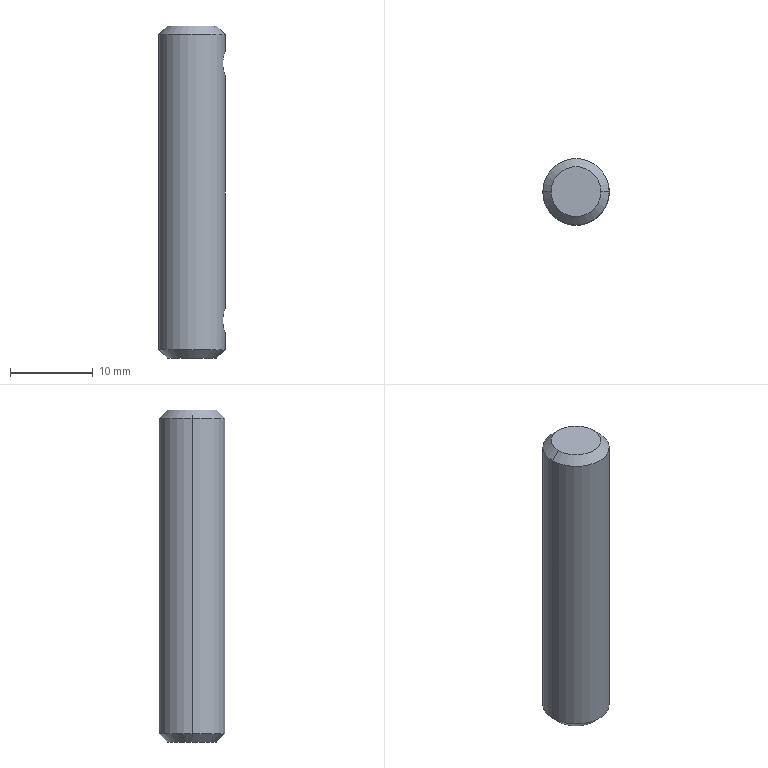Component | SolidWorks | ZTDJ-L-400-04-25-MaterialPortBagClamp-Axis6-1 | 1 solid | 16 faces | box 8 x 8 x 40 mm | volume 1928 mm3 | cone 8 | cylinder 6 | plane 2 | commonest cylinder face diameters 3 x4 8 x2 | material Alloy Steel
build123d program:
from build123d import *

# Parameters (mm, degrees)
SKETCH1_R                    = 4
BOSS_EXTRUDE1_DEPTH          = 20
F_3_0_3_DIAMETER_HOLE1_D     = 3
F_3_0_3_DIAMETER_HOLE1_DEPTH = 4
F_3_0_3_DIAMETER_HOLE1_TIP   = 0.9013
CHAMFER1_SIZE                = 1


with BuildPart() as part:
    # Sketch1 → Boss-Extrude1 (new, symmetric)
    with BuildSketch(Plane.XY):
        Circle(SKETCH1_R)
    extrude(amount=BOSS_EXTRUDE1_DEPTH, both=True)

    # 3.0 _3_ Diameter Hole1
    with Locations(Plane(origin=(4, 0, 0), x_dir=(0, 0, -1), z_dir=(1, 0, 0))):
        with Locations((-15.5, 0), (15.5, 0)):
            Hole(F_3_0_3_DIAMETER_HOLE1_D / 2, depth=F_3_0_3_DIAMETER_HOLE1_DEPTH)
            with Locations((0, 0, -(F_3_0_3_DIAMETER_HOLE1_DEPTH + F_3_0_3_DIAMETER_HOLE1_TIP / 2))):  # 118° drill point
                Cone(0, F_3_0_3_DIAMETER_HOLE1_D / 2, F_3_0_3_DIAMETER_HOLE1_TIP, mode=Mode.SUBTRACT)

    # Chamfer1
    chamfer1_edges = [part.edges().sort_by_distance(p)[0] for p in [
        (-4, 0, -20),
        (-4, 0, 20),
    ]]
    chamfer(chamfer1_edges, length=CHAMFER1_SIZE)


solid = part.part

# Placed as in the assembly
solid = solid.moved(Location((14.378, -64.673, 290), (0, 0, 0)))
STEP:
#1=COLOUR_RGB('',0.7922,0.8196,0.9333);
#2=FILL_AREA_STYLE_COLOUR('',#1);
#3=FILL_AREA_STYLE('',(#2));
#4=SURFACE_STYLE_FILL_AREA(#3);
#5=SURFACE_SIDE_STYLE('',(#4));
#6=SURFACE_STYLE_USAGE(.BOTH.,#5);
#7=PRESENTATION_STYLE_ASSIGNMENT((#6));
#8=CARTESIAN_POINT('',(0.6842,-2.546,12.205));
#9=VERTEX_POINT('',#8);
#10=CARTESIAN_POINT('',(0.448,-2.546,12.205));
#11=VERTEX_POINT('',#10);
#12=CARTESIAN_POINT('',(0.5661,-2.546,12.205));
#13=DIRECTION('',(0.,0.,1.));
#14=DIRECTION('',(1.,0.,0.));
#15=AXIS2_PLACEMENT_3D('',#12,#13,#14);
#16=CIRCLE('',#15,0.1181);
#17=EDGE_CURVE('',#9,#11,#16,.T.);
#18=ORIENTED_EDGE('',*,*,#17,.F.);
#19=CARTESIAN_POINT('',(0.7235,-2.546,12.165));
#20=VERTEX_POINT('',#19);
#21=CARTESIAN_POINT('',(0.6842,-2.546,12.205));
#22=DIRECTION('',(0.7071,0.,-0.7071));
#23=VECTOR('',#22,39.37);
#24=LINE('',#21,#23);
#25=EDGE_CURVE('',#9,#20,#24,.T.);
#26=ORIENTED_EDGE('',*,*,#25,.T.);
#27=CARTESIAN_POINT('',(0.4086,-2.546,12.165));
#28=VERTEX_POINT('',#27);
#29=CARTESIAN_POINT('',(0.5661,-2.546,12.165));
#30=DIRECTION('',(0.,0.,-1.));
#31=DIRECTION('',(1.,0.,0.));
#32=AXIS2_PLACEMENT_3D('',#29,#30,#31);
#33=CIRCLE('',#32,0.1575);
#34=EDGE_CURVE('',#28,#20,#33,.T.);
#35=ORIENTED_EDGE('',*,*,#34,.F.);
#36=CARTESIAN_POINT('',(0.448,-2.546,12.205));
#37=DIRECTION('',(-0.7071,0.,-0.7071));
#38=VECTOR('',#37,39.37);
#39=LINE('',#36,#38);
#40=EDGE_CURVE('',#11,#28,#39,.T.);
#41=ORIENTED_EDGE('',*,*,#40,.F.);
#42=EDGE_LOOP('',(#18,#26,#35,#41));
#43=FACE_OUTER_BOUND('',#42,.T.);
#44=CARTESIAN_POINT('',(0.5661,-2.546,12.205));
#45=DIRECTION('',(0.,0.,-1.));
#46=DIRECTION('',(-1.,0.,0.));
#47=AXIS2_PLACEMENT_3D('',#44,#45,#46);
#48=CONICAL_SURFACE('',#47,0.1181,0.7854);
#49=ADVANCED_FACE('',(#43),#48,.T.);
#50=CARTESIAN_POINT('',(0.448,-2.546,10.63));
#51=VERTEX_POINT('',#50);
#52=CARTESIAN_POINT('',(0.6842,-2.546,10.63));
#53=VERTEX_POINT('',#52);
#54=CARTESIAN_POINT('',(0.5661,-2.546,10.63));
#55=DIRECTION('',(0.,0.,-1.));
#56=DIRECTION('',(1.,0.,0.));
#57=AXIS2_PLACEMENT_3D('',#54,#55,#56);
#58=CIRCLE('',#57,0.1181);
#59=EDGE_CURVE('',#51,#53,#58,.T.);
#60=ORIENTED_EDGE('',*,*,#59,.F.);
#61=CARTESIAN_POINT('',(0.4086,-2.546,10.669));
#62=VERTEX_POINT('',#61);
#63=CARTESIAN_POINT('',(0.4086,-2.546,10.669));
#64=DIRECTION('',(-0.7071,0.,0.7071));
#65=VECTOR('',#64,39.37);
#66=LINE('',#63,#65);
#67=EDGE_CURVE('',#51,#62,#66,.T.);
#68=ORIENTED_EDGE('',*,*,#67,.T.);
#69=CARTESIAN_POINT('',(0.7235,-2.546,10.669));
#70=VERTEX_POINT('',#69);
#71=CARTESIAN_POINT('',(0.5661,-2.546,10.669));
#72=DIRECTION('',(0.,0.,1.));
#73=DIRECTION('',(1.,0.,0.));
#74=AXIS2_PLACEMENT_3D('',#71,#72,#73);
#75=CIRCLE('',#74,0.1575);
#76=EDGE_CURVE('',#70,#62,#75,.T.);
#77=ORIENTED_EDGE('',*,*,#76,.F.);
#78=CARTESIAN_POINT('',(0.7235,-2.546,10.669));
#79=DIRECTION('',(0.7071,0.,0.7071));
#80=VECTOR('',#79,39.37);
#81=LINE('',#78,#80);
#82=EDGE_CURVE('',#53,#70,#81,.T.);
#83=ORIENTED_EDGE('',*,*,#82,.F.);
#84=EDGE_LOOP('',(#60,#68,#77,#83));
#85=FACE_OUTER_BOUND('',#84,.T.);
#86=CARTESIAN_POINT('',(0.5661,-2.546,10.669));
#87=DIRECTION('',(0.,0.,1.));
#88=DIRECTION('',(1.,0.,0.));
#89=AXIS2_PLACEMENT_3D('',#86,#87,#88);
#90=CONICAL_SURFACE('',#89,0.1575,0.7854);
#91=ADVANCED_FACE('',(#85),#90,.T.);
#92=CARTESIAN_POINT('',(0.5306,-2.546,12.028));
#93=VERTEX_POINT('',#92);
#94=CARTESIAN_POINT('',(0.5661,-2.546,11.969));
#95=VERTEX_POINT('',#94);
#96=CARTESIAN_POINT('',(0.5661,-2.546,11.969));
#97=DIRECTION('',(0.515,0.,-0.8572));
#98=VECTOR('',#97,39.37);
#99=LINE('',#96,#98);
#100=EDGE_CURVE('',#93,#95,#99,.T.);
#101=ORIENTED_EDGE('',*,*,#100,.F.);
#102=CARTESIAN_POINT('',(0.5661,-2.546,12.087));
#103=VERTEX_POINT('',#102);
#104=CARTESIAN_POINT('',(0.5661,-2.546,12.087));
#105=DIRECTION('',(0.515,0.,0.8572));
#106=VECTOR('',#105,39.37);
#107=LINE('',#104,#106);
#108=EDGE_CURVE('',#93,#103,#107,.T.);
#109=ORIENTED_EDGE('',*,*,#108,.T.);
#110=CARTESIAN_POINT('',(0.5661,-2.546,12.028));
#111=DIRECTION('',(1.,0.,0.));
#112=DIRECTION('',(0.,0.,-1.));
#113=AXIS2_PLACEMENT_3D('',#110,#111,#112);
#114=CIRCLE('',#113,0.05906);
#115=EDGE_CURVE('',#103,#95,#114,.T.);
#116=ORIENTED_EDGE('',*,*,#115,.T.);
#117=EDGE_LOOP('',(#101,#109,#116));
#118=FACE_OUTER_BOUND('',#117,.T.);
#119=CARTESIAN_POINT('',(0.5661,-2.546,12.028));
#120=DIRECTION('',(1.,0.,0.));
#121=DIRECTION('',(0.,0.,-1.));
#122=AXIS2_PLACEMENT_3D('',#119,#120,#121);
#123=CONICAL_SURFACE('',#122,0.05906,1.03);
#124=ADVANCED_FACE('',(#118),#123,.F.);
#125=ORIENTED_EDGE('',*,*,#115,.F.);
#126=CARTESIAN_POINT('',(0.7235,-2.546,12.087));
#127=VERTEX_POINT('',#126);
#128=CARTESIAN_POINT('',(0.7235,-2.546,12.087));
#129=DIRECTION('',(1.,0.,0.));
#130=VECTOR('',#129,39.37);
#131=LINE('',#128,#130);
#132=EDGE_CURVE('',#103,#127,#131,.T.);
#133=ORIENTED_EDGE('',*,*,#132,.T.);
#134=CARTESIAN_POINT('',(0.7235,-2.546,11.969));
#135=VERTEX_POINT('',#134);
#136=CARTESIAN_POINT('',(0.7235,-2.546,11.969));
#137=CARTESIAN_POINT('',(0.7235,-2.55,11.969));
#138=CARTESIAN_POINT('',(0.7234,-2.554,11.969));
#139=CARTESIAN_POINT('',(0.7228,-2.562,11.97));
#140=CARTESIAN_POINT('',(0.7224,-2.565,11.972));
#141=CARTESIAN_POINT('',(0.7209,-2.576,11.976));
#142=CARTESIAN_POINT('',(0.7194,-2.583,11.98));
#143=CARTESIAN_POINT('',(0.7164,-2.593,11.991));
#144=CARTESIAN_POINT('',(0.7149,-2.598,11.998));
#145=CARTESIAN_POINT('',(0.7133,-2.602,12.008));
#146=CARTESIAN_POINT('',(0.7128,-2.603,12.012));
#147=CARTESIAN_POINT('',(0.7122,-2.605,12.02));
#148=CARTESIAN_POINT('',(0.7121,-2.605,12.024));
#149=CARTESIAN_POINT('',(0.7121,-2.605,12.031));
#150=CARTESIAN_POINT('',(0.7122,-2.605,12.035));
#151=CARTESIAN_POINT('',(0.7128,-2.603,12.043));
#152=CARTESIAN_POINT('',(0.7133,-2.602,12.047));
#153=CARTESIAN_POINT('',(0.7144,-2.599,12.054));
#154=CARTESIAN_POINT('',(0.715,-2.597,12.057));
#155=CARTESIAN_POINT('',(0.7164,-2.593,12.064));
#156=CARTESIAN_POINT('',(0.7172,-2.591,12.067));
#157=CARTESIAN_POINT('',(0.7187,-2.585,12.072));
#158=CARTESIAN_POINT('',(0.7194,-2.582,12.074));
#159=CARTESIAN_POINT('',(0.7208,-2.576,12.079));
#160=CARTESIAN_POINT('',(0.7214,-2.572,12.081));
#161=CARTESIAN_POINT('',(0.7229,-2.562,12.085));
#162=CARTESIAN_POINT('',(0.7235,-2.554,12.087));
#163=CARTESIAN_POINT('',(0.7235,-2.546,12.087));
#164=B_SPLINE_CURVE_WITH_KNOTS('',3,(#136,#137,#138,#139,#140,#141,#142,#143,#144,#145,#146,#147,#148,#149,#150,#151,#152,#153,#154,#155,#156,#157,#158,#159,#160,#161,#162,#163),.UNSPECIFIED.,.F.,.F.,(4,2,2,2,2,2,2,2,2,2,2,2,2,4),(0.,0.0002958,0.0005917,0.001183,0.001775,0.002071,0.002367,0.002663,0.002958,0.003254,0.00355,0.003846,0.004142,0.004733),.UNSPECIFIED.);
#165=EDGE_CURVE('',#135,#127,#164,.T.);
#166=ORIENTED_EDGE('',*,*,#165,.F.);
#167=CARTESIAN_POINT('',(0.7235,-2.546,11.969));
#168=DIRECTION('',(1.,0.,0.));
#169=VECTOR('',#168,39.37);
#170=LINE('',#167,#169);
#171=EDGE_CURVE('',#95,#135,#170,.T.);
#172=ORIENTED_EDGE('',*,*,#171,.F.);
#173=EDGE_LOOP('',(#125,#133,#166,#172));
#174=FACE_OUTER_BOUND('',#173,.T.);
#175=CARTESIAN_POINT('',(0.7235,-2.546,12.028));
#176=DIRECTION('',(1.,0.,0.));
#177=DIRECTION('',(0.,0.,-1.));
#178=AXIS2_PLACEMENT_3D('',#175,#176,#177);
#179=CYLINDRICAL_SURFACE('',#178,0.05906);
#180=ADVANCED_FACE('',(#174),#179,.F.);
#181=CARTESIAN_POINT('',(0.5306,-2.546,10.807));
#182=VERTEX_POINT('',#181);
#183=CARTESIAN_POINT('',(0.5661,-2.546,10.748));
#184=VERTEX_POINT('',#183);
#185=CARTESIAN_POINT('',(0.5661,-2.546,10.748));
#186=DIRECTION('',(0.515,0.,-0.8572));
#187=VECTOR('',#186,39.37);
#188=LINE('',#185,#187);
#189=EDGE_CURVE('',#182,#184,#188,.T.);
#190=ORIENTED_EDGE('',*,*,#189,.F.);
#191=CARTESIAN_POINT('',(0.5661,-2.546,10.866));
#192=VERTEX_POINT('',#191);
#193=CARTESIAN_POINT('',(0.5661,-2.546,10.866));
#194=DIRECTION('',(0.515,0.,0.8572));
#195=VECTOR('',#194,39.37);
#196=LINE('',#193,#195);
#197=EDGE_CURVE('',#182,#192,#196,.T.);
#198=ORIENTED_EDGE('',*,*,#197,.T.);
#199=CARTESIAN_POINT('',(0.5661,-2.546,10.807));
#200=DIRECTION('',(1.,0.,0.));
#201=DIRECTION('',(0.,0.,-1.));
#202=AXIS2_PLACEMENT_3D('',#199,#200,#201);
#203=CIRCLE('',#202,0.05906);
#204=EDGE_CURVE('',#192,#184,#203,.T.);
#205=ORIENTED_EDGE('',*,*,#204,.T.);
#206=EDGE_LOOP('',(#190,#198,#205));
#207=FACE_OUTER_BOUND('',#206,.T.);
#208=CARTESIAN_POINT('',(0.5661,-2.546,10.807));
#209=DIRECTION('',(1.,0.,0.));
#210=DIRECTION('',(0.,0.,-1.));
#211=AXIS2_PLACEMENT_3D('',#208,#209,#210);
#212=CONICAL_SURFACE('',#211,0.05906,1.03);
#213=ADVANCED_FACE('',(#207),#212,.F.);
#214=ORIENTED_EDGE('',*,*,#204,.F.);
#215=CARTESIAN_POINT('',(0.7235,-2.546,10.866));
#216=VERTEX_POINT('',#215);
#217=CARTESIAN_POINT('',(0.7235,-2.546,10.866));
#218=DIRECTION('',(1.,0.,0.));
#219=VECTOR('',#218,39.37);
#220=LINE('',#217,#219);
#221=EDGE_CURVE('',#192,#216,#220,.T.);
#222=ORIENTED_EDGE('',*,*,#221,.T.);
#223=CARTESIAN_POINT('',(0.7235,-2.546,10.748));
#224=VERTEX_POINT('',#223);
#225=CARTESIAN_POINT('',(0.7235,-2.546,10.748));
#226=CARTESIAN_POINT('',(0.7235,-2.55,10.748));
#227=CARTESIAN_POINT('',(0.7234,-2.554,10.748));
#228=CARTESIAN_POINT('',(0.7228,-2.562,10.75));
#229=CARTESIAN_POINT('',(0.7224,-2.565,10.751));
#230=CARTESIAN_POINT('',(0.7209,-2.576,10.756));
#231=CARTESIAN_POINT('',(0.7194,-2.583,10.76));
#232=CARTESIAN_POINT('',(0.7164,-2.593,10.771));
#233=CARTESIAN_POINT('',(0.7149,-2.598,10.777));
#234=CARTESIAN_POINT('',(0.7133,-2.602,10.788));
#235=CARTESIAN_POINT('',(0.7128,-2.603,10.792));
#236=CARTESIAN_POINT('',(0.7122,-2.605,10.799));
#237=CARTESIAN_POINT('',(0.7121,-2.605,10.803));
#238=CARTESIAN_POINT('',(0.7121,-2.605,10.811));
#239=CARTESIAN_POINT('',(0.7122,-2.605,10.815));
#240=CARTESIAN_POINT('',(0.7128,-2.603,10.823));
#241=CARTESIAN_POINT('',(0.7133,-2.602,10.826));
#242=CARTESIAN_POINT('',(0.7144,-2.599,10.833));
#243=CARTESIAN_POINT('',(0.715,-2.597,10.837));
#244=CARTESIAN_POINT('',(0.7164,-2.593,10.843));
#245=CARTESIAN_POINT('',(0.7172,-2.591,10.846));
#246=CARTESIAN_POINT('',(0.7187,-2.585,10.852));
#247=CARTESIAN_POINT('',(0.7194,-2.582,10.854));
#248=CARTESIAN_POINT('',(0.7208,-2.576,10.858));
#249=CARTESIAN_POINT('',(0.7214,-2.572,10.86));
#250=CARTESIAN_POINT('',(0.7229,-2.562,10.865));
#251=CARTESIAN_POINT('',(0.7235,-2.554,10.866));
#252=CARTESIAN_POINT('',(0.7235,-2.546,10.866));
#253=B_SPLINE_CURVE_WITH_KNOTS('',3,(#225,#226,#227,#228,#229,#230,#231,#232,#233,#234,#235,#236,#237,#238,#239,#240,#241,#242,#243,#244,#245,#246,#247,#248,#249,#250,#251,#252),.UNSPECIFIED.,.F.,.F.,(4,2,2,2,2,2,2,2,2,2,2,2,2,4),(0.,0.0002958,0.0005917,0.001183,0.001775,0.002071,0.002367,0.002663,0.002958,0.003254,0.00355,0.003846,0.004142,0.004733),.UNSPECIFIED.);
#254=EDGE_CURVE('',#224,#216,#253,.T.);
#255=ORIENTED_EDGE('',*,*,#254,.F.);
#256=CARTESIAN_POINT('',(0.7235,-2.546,10.748));
#257=DIRECTION('',(1.,0.,0.));
#258=VECTOR('',#257,39.37);
#259=LINE('',#256,#258);
#260=EDGE_CURVE('',#184,#224,#259,.T.);
#261=ORIENTED_EDGE('',*,*,#260,.F.);
#262=EDGE_LOOP('',(#214,#222,#255,#261));
#263=FACE_OUTER_BOUND('',#262,.T.);
#264=CARTESIAN_POINT('',(0.7235,-2.546,10.807));
#265=DIRECTION('',(1.,0.,0.));
#266=DIRECTION('',(0.,0.,-1.));
#267=AXIS2_PLACEMENT_3D('',#264,#265,#266);
#268=CYLINDRICAL_SURFACE('',#267,0.05906);
#269=ADVANCED_FACE('',(#263),#268,.F.);
#270=ORIENTED_EDGE('',*,*,#34,.T.);
#271=CARTESIAN_POINT('',(0.7235,-2.546,12.205));
#272=DIRECTION('',(0.,0.,-1.));
#273=VECTOR('',#272,39.37);
#274=LINE('',#271,#273);
#275=EDGE_CURVE('',#20,#127,#274,.T.);
#276=ORIENTED_EDGE('',*,*,#275,.T.);
#277=CARTESIAN_POINT('',(0.7235,-2.546,12.087));
#278=CARTESIAN_POINT('',(0.7235,-2.538,12.087));
#279=CARTESIAN_POINT('',(0.7229,-2.531,12.085));
#280=CARTESIAN_POINT('',(0.7214,-2.52,12.081));
#281=CARTESIAN_POINT('',(0.7207,-2.516,12.079));
#282=CARTESIAN_POINT('',(0.7194,-2.51,12.074));
#283=CARTESIAN_POINT('',(0.7187,-2.507,12.072));
#284=CARTESIAN_POINT('',(0.7164,-2.499,12.064));
#285=CARTESIAN_POINT('',(0.7149,-2.495,12.057));
#286=CARTESIAN_POINT('',(0.7133,-2.49,12.047));
#287=CARTESIAN_POINT('',(0.7128,-2.489,12.043));
#288=CARTESIAN_POINT('',(0.7122,-2.488,12.035));
#289=CARTESIAN_POINT('',(0.7121,-2.487,12.031));
#290=CARTESIAN_POINT('',(0.7121,-2.487,12.02));
#291=CARTESIAN_POINT('',(0.7127,-2.489,12.012));
#292=CARTESIAN_POINT('',(0.7149,-2.495,11.998));
#293=CARTESIAN_POINT('',(0.7164,-2.499,11.991));
#294=CARTESIAN_POINT('',(0.7187,-2.507,11.983));
#295=CARTESIAN_POINT('',(0.7194,-2.51,11.981));
#296=CARTESIAN_POINT('',(0.7208,-2.517,11.976));
#297=CARTESIAN_POINT('',(0.7214,-2.52,11.975));
#298=CARTESIAN_POINT('',(0.7229,-2.531,11.97));
#299=CARTESIAN_POINT('',(0.7235,-2.538,11.969));
#300=CARTESIAN_POINT('',(0.7235,-2.546,11.969));
#301=B_SPLINE_CURVE_WITH_KNOTS('',3,(#277,#278,#279,#280,#281,#282,#283,#284,#285,#286,#287,#288,#289,#290,#291,#292,#293,#294,#295,#296,#297,#298,#299,#300),.UNSPECIFIED.,.F.,.F.,(4,2,2,2,2,2,2,2,2,2,2,4),(0.004733,0.005325,0.005621,0.005916,0.006508,0.006804,0.0071,0.007691,0.008283,0.008578,0.008874,0.009466),.UNSPECIFIED.);
#302=EDGE_CURVE('',#127,#135,#301,.T.);
#303=ORIENTED_EDGE('',*,*,#302,.T.);
#304=CARTESIAN_POINT('',(0.7235,-2.546,12.205));
#305=DIRECTION('',(0.,0.,-1.));
#306=VECTOR('',#305,39.37);
#307=LINE('',#304,#306);
#308=EDGE_CURVE('',#135,#216,#307,.T.);
#309=ORIENTED_EDGE('',*,*,#308,.T.);
#310=CARTESIAN_POINT('',(0.7235,-2.546,10.866));
#311=CARTESIAN_POINT('',(0.7235,-2.538,10.866));
#312=CARTESIAN_POINT('',(0.7229,-2.531,10.865));
#313=CARTESIAN_POINT('',(0.7214,-2.52,10.86));
#314=CARTESIAN_POINT('',(0.7207,-2.516,10.858));
#315=CARTESIAN_POINT('',(0.7194,-2.51,10.854));
#316=CARTESIAN_POINT('',(0.7187,-2.507,10.852));
#317=CARTESIAN_POINT('',(0.7164,-2.499,10.843));
#318=CARTESIAN_POINT('',(0.7149,-2.495,10.837));
#319=CARTESIAN_POINT('',(0.7133,-2.49,10.826));
#320=CARTESIAN_POINT('',(0.7128,-2.489,10.823));
#321=CARTESIAN_POINT('',(0.7122,-2.488,10.815));
#322=CARTESIAN_POINT('',(0.7121,-2.487,10.811));
#323=CARTESIAN_POINT('',(0.7121,-2.487,10.799));
#324=CARTESIAN_POINT('',(0.7127,-2.489,10.791));
#325=CARTESIAN_POINT('',(0.7149,-2.495,10.777));
#326=CARTESIAN_POINT('',(0.7164,-2.499,10.771));
#327=CARTESIAN_POINT('',(0.7187,-2.507,10.763));
#328=CARTESIAN_POINT('',(0.7194,-2.51,10.76));
#329=CARTESIAN_POINT('',(0.7208,-2.517,10.756));
#330=CARTESIAN_POINT('',(0.7214,-2.52,10.754));
#331=CARTESIAN_POINT('',(0.7229,-2.531,10.75));
#332=CARTESIAN_POINT('',(0.7235,-2.538,10.748));
#333=CARTESIAN_POINT('',(0.7235,-2.546,10.748));
#334=B_SPLINE_CURVE_WITH_KNOTS('',3,(#310,#311,#312,#313,#314,#315,#316,#317,#318,#319,#320,#321,#322,#323,#324,#325,#326,#327,#328,#329,#330,#331,#332,#333),.UNSPECIFIED.,.F.,.F.,(4,2,2,2,2,2,2,2,2,2,2,4),(0.004733,0.005325,0.005621,0.005916,0.006508,0.006804,0.0071,0.007691,0.008283,0.008578,0.008874,0.009466),.UNSPECIFIED.);
#335=EDGE_CURVE('',#216,#224,#334,.T.);
#336=ORIENTED_EDGE('',*,*,#335,.T.);
#337=CARTESIAN_POINT('',(0.7235,-2.546,12.205));
#338=DIRECTION('',(0.,0.,-1.));
#339=VECTOR('',#338,39.37);
#340=LINE('',#337,#339);
#341=EDGE_CURVE('',#224,#70,#340,.T.);
#342=ORIENTED_EDGE('',*,*,#341,.T.);
#343=ORIENTED_EDGE('',*,*,#76,.T.);
#344=CARTESIAN_POINT('',(0.4086,-2.546,12.205));
#345=DIRECTION('',(0.,0.,-1.));
#346=VECTOR('',#345,39.37);
#347=LINE('',#344,#346);
#348=EDGE_CURVE('',#28,#62,#347,.T.);
#349=ORIENTED_EDGE('',*,*,#348,.F.);
#350=EDGE_LOOP('',(#270,#276,#303,#309,#336,#342,#343,#349));
#351=FACE_OUTER_BOUND('',#350,.T.);
#352=CARTESIAN_POINT('',(0.5661,-2.546,12.205));
#353=DIRECTION('',(0.,0.,-1.));
#354=DIRECTION('',(-1.,0.,0.));
#355=AXIS2_PLACEMENT_3D('',#352,#353,#354);
#356=CYLINDRICAL_SURFACE('',#355,0.1575);
#357=ADVANCED_FACE('',(#351),#356,.T.);
#358=ORIENTED_EDGE('',*,*,#275,.F.);
#359=CARTESIAN_POINT('',(0.5661,-2.546,12.165));
#360=DIRECTION('',(0.,0.,-1.));
#361=DIRECTION('',(1.,0.,0.));
#362=AXIS2_PLACEMENT_3D('',#359,#360,#361);
#363=CIRCLE('',#362,0.1575);
#364=EDGE_CURVE('',#20,#28,#363,.T.);
#365=ORIENTED_EDGE('',*,*,#364,.T.);
#366=ORIENTED_EDGE('',*,*,#348,.T.);
#367=CARTESIAN_POINT('',(0.5661,-2.546,10.669));
#368=DIRECTION('',(0.,0.,1.));
#369=DIRECTION('',(1.,0.,0.));
#370=AXIS2_PLACEMENT_3D('',#367,#368,#369);
#371=CIRCLE('',#370,0.1575);
#372=EDGE_CURVE('',#62,#70,#371,.T.);
#373=ORIENTED_EDGE('',*,*,#372,.T.);
#374=ORIENTED_EDGE('',*,*,#341,.F.);
#375=ORIENTED_EDGE('',*,*,#254,.T.);
#376=ORIENTED_EDGE('',*,*,#308,.F.);
#377=ORIENTED_EDGE('',*,*,#165,.T.);
#378=EDGE_LOOP('',(#358,#365,#366,#373,#374,#375,#376,#377));
#379=FACE_OUTER_BOUND('',#378,.T.);
#380=CARTESIAN_POINT('',(0.5661,-2.546,12.205));
#381=DIRECTION('',(0.,0.,-1.));
#382=DIRECTION('',(-1.,0.,0.));
#383=AXIS2_PLACEMENT_3D('',#380,#381,#382);
#384=CYLINDRICAL_SURFACE('',#383,0.1575);
#385=ADVANCED_FACE('',(#379),#384,.T.);
#386=CARTESIAN_POINT('',(0.5661,-2.546,12.205));
#387=DIRECTION('',(0.,0.,1.));
#388=DIRECTION('',(1.,0.,0.));
#389=AXIS2_PLACEMENT_3D('',#386,#387,#388);
#390=CIRCLE('',#389,0.1181);
#391=EDGE_CURVE('',#11,#9,#390,.T.);
#392=ORIENTED_EDGE('',*,*,#391,.T.);
#393=ORIENTED_EDGE('',*,*,#17,.T.);
#394=EDGE_LOOP('',(#392,#393));
#395=FACE_OUTER_BOUND('',#394,.T.);
#396=CARTESIAN_POINT('',(0.5661,-2.546,12.205));
#397=DIRECTION('',(0.,0.,1.));
#398=DIRECTION('',(1.,0.,0.));
#399=AXIS2_PLACEMENT_3D('',#396,#397,#398);
#400=PLANE('',#399);
#401=ADVANCED_FACE('',(#395),#400,.T.);
#402=CARTESIAN_POINT('',(0.5661,-2.546,10.63));
#403=DIRECTION('',(0.,0.,-1.));
#404=DIRECTION('',(1.,0.,0.));
#405=AXIS2_PLACEMENT_3D('',#402,#403,#404);
#406=CIRCLE('',#405,0.1181);
#407=EDGE_CURVE('',#53,#51,#406,.T.);
#408=ORIENTED_EDGE('',*,*,#407,.T.);
#409=ORIENTED_EDGE('',*,*,#59,.T.);
#410=EDGE_LOOP('',(#408,#409));
#411=FACE_OUTER_BOUND('',#410,.T.);
#412=CARTESIAN_POINT('',(0.5661,-2.546,10.63));
#413=DIRECTION('',(0.,0.,1.));
#414=DIRECTION('',(1.,0.,0.));
#415=AXIS2_PLACEMENT_3D('',#412,#413,#414);
#416=PLANE('',#415);
#417=ADVANCED_FACE('',(#411),#416,.F.);
#418=ORIENTED_EDGE('',*,*,#221,.F.);
#419=CARTESIAN_POINT('',(0.5661,-2.546,10.807));
#420=DIRECTION('',(1.,0.,0.));
#421=DIRECTION('',(0.,0.,-1.));
#422=AXIS2_PLACEMENT_3D('',#419,#420,#421);
#423=CIRCLE('',#422,0.05906);
#424=EDGE_CURVE('',#184,#192,#423,.T.);
#425=ORIENTED_EDGE('',*,*,#424,.F.);
#426=ORIENTED_EDGE('',*,*,#260,.T.);
#427=ORIENTED_EDGE('',*,*,#335,.F.);
#428=EDGE_LOOP('',(#418,#425,#426,#427));
#429=FACE_OUTER_BOUND('',#428,.T.);
#430=CARTESIAN_POINT('',(0.7235,-2.546,10.807));
#431=DIRECTION('',(1.,0.,0.));
#432=DIRECTION('',(0.,0.,-1.));
#433=AXIS2_PLACEMENT_3D('',#430,#431,#432);
#434=CYLINDRICAL_SURFACE('',#433,0.05906);
#435=ADVANCED_FACE('',(#429),#434,.F.);
#436=ORIENTED_EDGE('',*,*,#197,.F.);
#437=ORIENTED_EDGE('',*,*,#189,.T.);
#438=ORIENTED_EDGE('',*,*,#424,.T.);
#439=EDGE_LOOP('',(#436,#437,#438));
#440=FACE_OUTER_BOUND('',#439,.T.);
#441=CARTESIAN_POINT('',(0.5661,-2.546,10.807));
#442=DIRECTION('',(1.,0.,0.));
#443=DIRECTION('',(0.,0.,-1.));
#444=AXIS2_PLACEMENT_3D('',#441,#442,#443);
#445=CONICAL_SURFACE('',#444,0.05906,1.03);
#446=ADVANCED_FACE('',(#440),#445,.F.);
#447=ORIENTED_EDGE('',*,*,#132,.F.);
#448=CARTESIAN_POINT('',(0.5661,-2.546,12.028));
#449=DIRECTION('',(1.,0.,0.));
#450=DIRECTION('',(0.,0.,-1.));
#451=AXIS2_PLACEMENT_3D('',#448,#449,#450);
#452=CIRCLE('',#451,0.05906);
#453=EDGE_CURVE('',#95,#103,#452,.T.);
#454=ORIENTED_EDGE('',*,*,#453,.F.);
#455=ORIENTED_EDGE('',*,*,#171,.T.);
#456=ORIENTED_EDGE('',*,*,#302,.F.);
#457=EDGE_LOOP('',(#447,#454,#455,#456));
#458=FACE_OUTER_BOUND('',#457,.T.);
#459=CARTESIAN_POINT('',(0.7235,-2.546,12.028));
#460=DIRECTION('',(1.,0.,0.));
#461=DIRECTION('',(0.,0.,-1.));
#462=AXIS2_PLACEMENT_3D('',#459,#460,#461);
#463=CYLINDRICAL_SURFACE('',#462,0.05906);
#464=ADVANCED_FACE('',(#458),#463,.F.);
#465=ORIENTED_EDGE('',*,*,#108,.F.);
#466=ORIENTED_EDGE('',*,*,#100,.T.);
#467=ORIENTED_EDGE('',*,*,#453,.T.);
#468=EDGE_LOOP('',(#465,#466,#467));
#469=FACE_OUTER_BOUND('',#468,.T.);
#470=CARTESIAN_POINT('',(0.5661,-2.546,12.028));
#471=DIRECTION('',(1.,0.,0.));
#472=DIRECTION('',(0.,0.,-1.));
#473=AXIS2_PLACEMENT_3D('',#470,#471,#472);
#474=CONICAL_SURFACE('',#473,0.05906,1.03);
#475=ADVANCED_FACE('',(#469),#474,.F.);
#476=ORIENTED_EDGE('',*,*,#67,.F.);
#477=ORIENTED_EDGE('',*,*,#407,.F.);
#478=ORIENTED_EDGE('',*,*,#82,.T.);
#479=ORIENTED_EDGE('',*,*,#372,.F.);
#480=EDGE_LOOP('',(#476,#477,#478,#479));
#481=FACE_OUTER_BOUND('',#480,.T.);
#482=CARTESIAN_POINT('',(0.5661,-2.546,10.669));
#483=DIRECTION('',(0.,0.,1.));
#484=DIRECTION('',(1.,0.,0.));
#485=AXIS2_PLACEMENT_3D('',#482,#483,#484);
#486=CONICAL_SURFACE('',#485,0.1575,0.7854);
#487=ADVANCED_FACE('',(#481),#486,.T.);
#488=ORIENTED_EDGE('',*,*,#25,.F.);
#489=ORIENTED_EDGE('',*,*,#391,.F.);
#490=ORIENTED_EDGE('',*,*,#40,.T.);
#491=ORIENTED_EDGE('',*,*,#364,.F.);
#492=EDGE_LOOP('',(#488,#489,#490,#491));
#493=FACE_OUTER_BOUND('',#492,.T.);
#494=CARTESIAN_POINT('',(0.5661,-2.546,12.205));
#495=DIRECTION('',(0.,0.,-1.));
#496=DIRECTION('',(-1.,0.,0.));
#497=AXIS2_PLACEMENT_3D('',#494,#495,#496);
#498=CONICAL_SURFACE('',#497,0.1181,0.7854);
#499=ADVANCED_FACE('',(#493),#498,.T.);
#500=CLOSED_SHELL('',(#49,#91,#124,#180,#213,#269,#357,#385,#401,#417,#435,#446,#464,#475,#487,#499));
#501=MANIFOLD_SOLID_BREP('',#500);
#502=STYLED_ITEM('',(#7),#501);
#503=(LENGTH_UNIT()NAMED_UNIT(*)SI_UNIT($,.METRE.));
#504=LENGTH_MEASURE_WITH_UNIT(LENGTH_MEASURE(0.0254),#503);
#505=DIMENSIONAL_EXPONENTS(1.,0.,0.,0.,0.,0.,0.);
#506=(CONVERSION_BASED_UNIT('',#504)LENGTH_UNIT()NAMED_UNIT(#505));
#507=UNCERTAINTY_MEASURE_WITH_UNIT(LENGTH_MEASURE(0.00001),#506,'','');
#508=(NAMED_UNIT(*)PLANE_ANGLE_UNIT()SI_UNIT($,.RADIAN.));
#509=(NAMED_UNIT(*)SI_UNIT($,.STERADIAN.)SOLID_ANGLE_UNIT());
#510=(GEOMETRIC_REPRESENTATION_CONTEXT(3)GLOBAL_UNCERTAINTY_ASSIGNED_CONTEXT((#507))GLOBAL_UNIT_ASSIGNED_CONTEXT((#506,#508,#509))REPRESENTATION_CONTEXT('',''));
#511=MECHANICAL_DESIGN_GEOMETRIC_PRESENTATION_REPRESENTATION('',(#502),#510);
#512=CARTESIAN_POINT('',(0.,0.,0.));
#513=DIRECTION('',(0.,0.,1.));
#514=DIRECTION('',(1.,0.,0.));
#515=AXIS2_PLACEMENT_3D('',#512,#513,#514);
#516=(LENGTH_UNIT()NAMED_UNIT(*)SI_UNIT($,.METRE.));
#517=LENGTH_MEASURE_WITH_UNIT(LENGTH_MEASURE(0.0254),#516);
#518=DIMENSIONAL_EXPONENTS(1.,0.,0.,0.,0.,0.,0.);
#519=(CONVERSION_BASED_UNIT('',#517)LENGTH_UNIT()NAMED_UNIT(#518));
#520=UNCERTAINTY_MEASURE_WITH_UNIT(LENGTH_MEASURE(0.00001),#519,'','');
#521=(NAMED_UNIT(*)PLANE_ANGLE_UNIT()SI_UNIT($,.RADIAN.));
#522=(NAMED_UNIT(*)SI_UNIT($,.STERADIAN.)SOLID_ANGLE_UNIT());
#523=(GEOMETRIC_REPRESENTATION_CONTEXT(3)GLOBAL_UNCERTAINTY_ASSIGNED_CONTEXT((#520))GLOBAL_UNIT_ASSIGNED_CONTEXT((#519,#521,#522))REPRESENTATION_CONTEXT('',''));
#524=ADVANCED_BREP_SHAPE_REPRESENTATION('',(#501,#515),#523);
#525=PRESENTATION_LAYER_ASSIGNMENT('','',(#502));